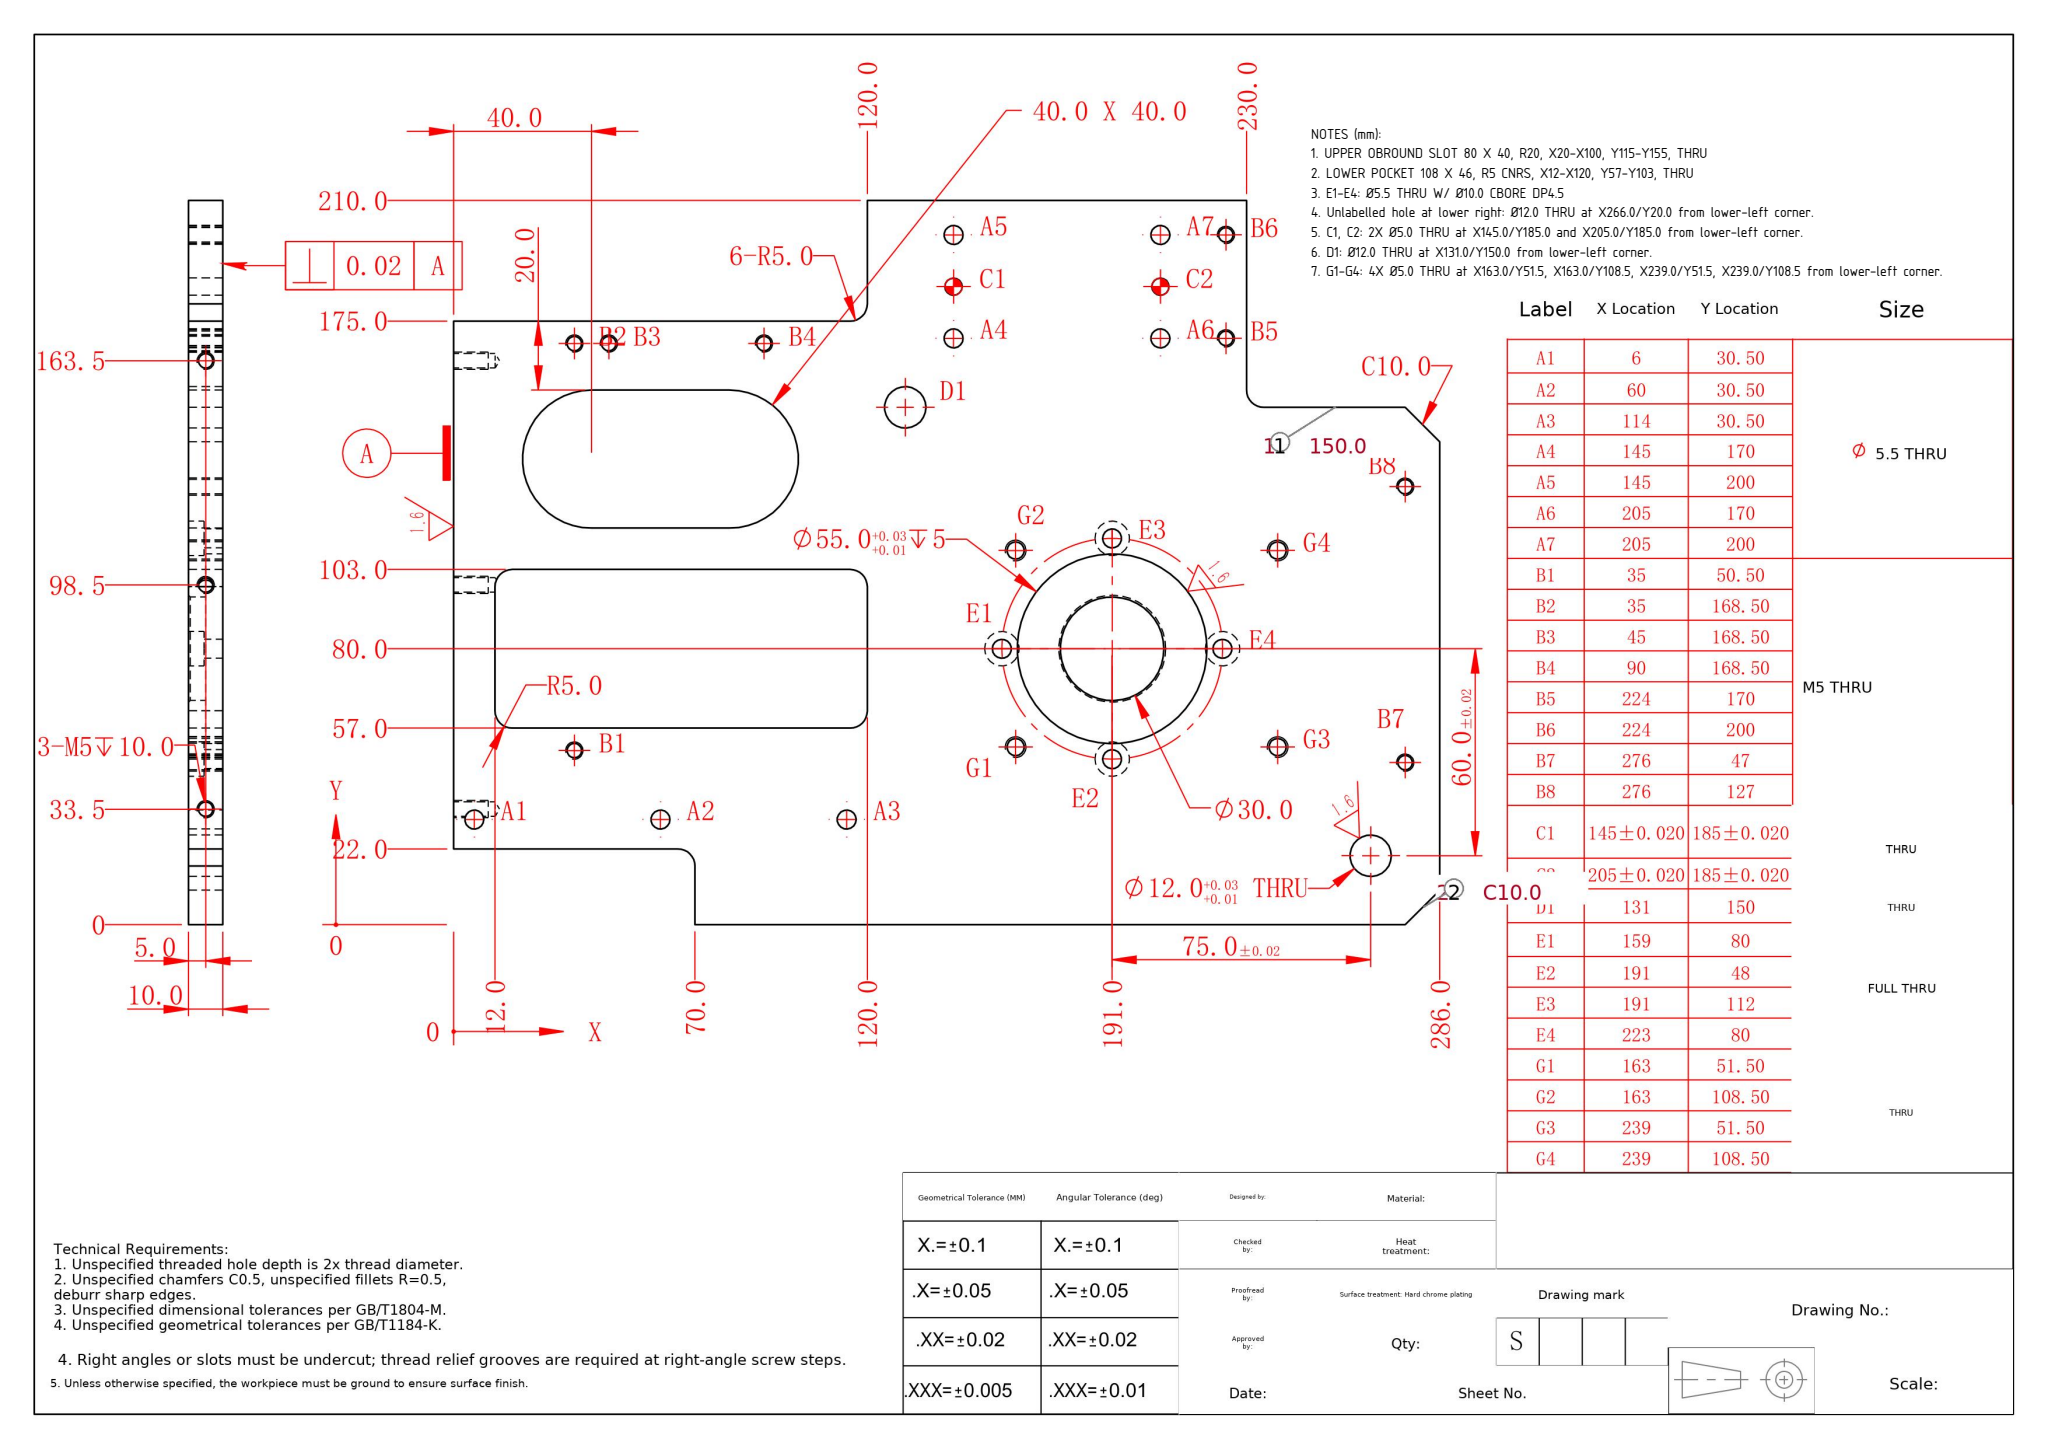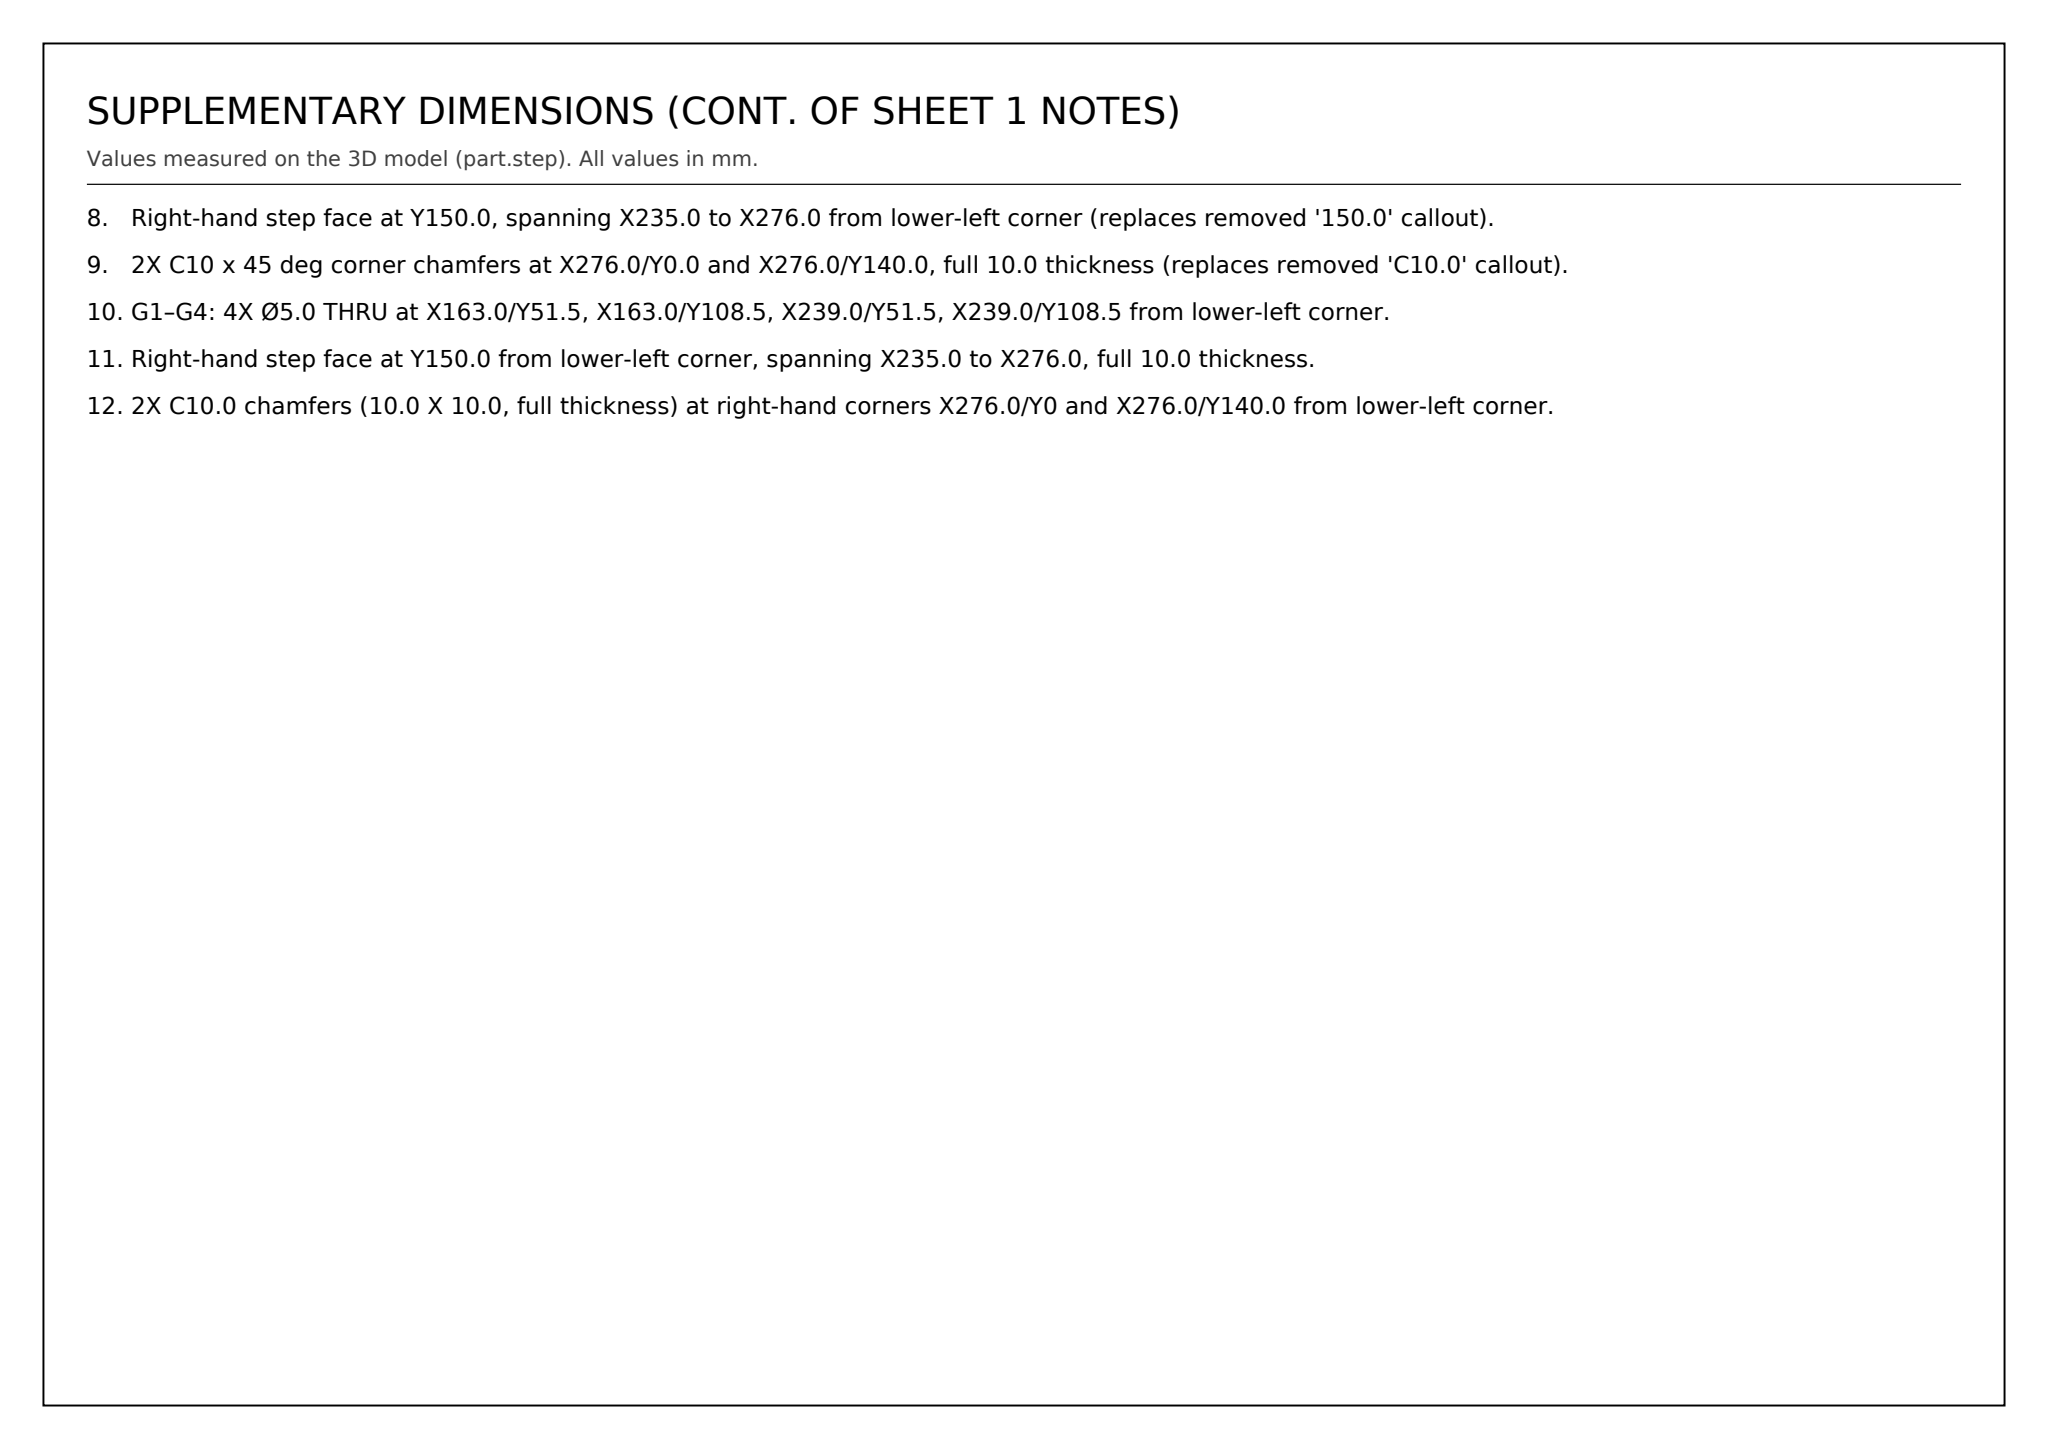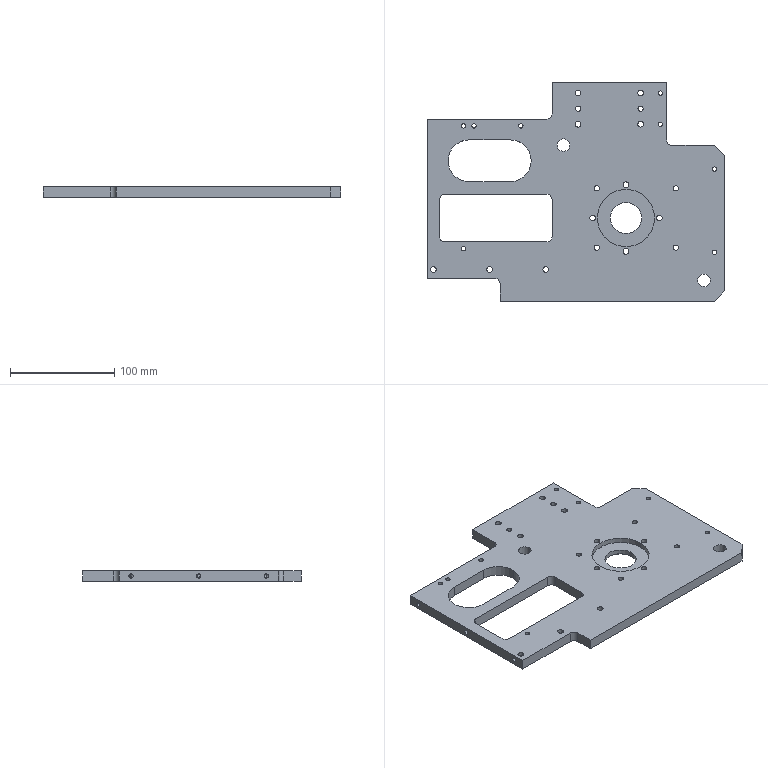Part | SolidWorks | mm | 1 solid | 116 faces | box 286 x 210 x 10 mm | volume 406665 mm3 | cylinder 82 | plane 25 | cone 9 | commonest cylinder face diameters 5.5 x22 4.2 x22 10 x15 5 x12 12 x4 40 x3 55 x2 30 x2
Drawing notes:
UPPER OBROUND SLOT 80 X 40, R20, X20-X100, Y115-Y155, THRU | from the solid: Ø40 cyls @ (40,135)&(80,135) len 10; planes y=115, y=155
LOWER POCKET 108 X 46, R5 CNRS, X12-X120, Y57-Y103, THRU | from the solid: R5 cnr cyls @ (17,62)(17,98)(115,62)(115,98) len 10; planes x=12/120, y=57/103
E1-E4: Ø5.5 THRU W/ Ø10.0 CBORE DP4.5 | from the solid: Ø5.5 len 5.5 and Ø10 len 4.5 coaxial @ (159,80)(191,48)(191,112)(223,80)
Unlabelled hole at lower right: Ø12.0 THRU at X266.0/Y20.0 from lower-left corner. | from the solid: cylinder dia 12.0, axis z, pos [266.0,20.0], length 10.0 = full 10.0 thk
C1, C2: 2X Ø5.0 THRU at X145.0/Y185.0 and X205.0/Y185.0 from lower-left corner. | from the solid: cylinders hole/bore dia 5.0, axis z at [145.0,185.0] and [205.0,185.0], from 0.0 to 10.0 (full 10 mm thickness)
D1: Ø12.0 THRU at X131.0/Y150.0 from lower-left corner. | from the solid: cylinders hole/bore dia 12.0, axis z at [131.0,150.0], from 0.0 to 10.0
G1-G4: 4X Ø5.0 THRU at X163.0/Y51.5, X163.0/Y108.5, X239.0/Y51.5, X239.0/Y108.5 from lower-left corner. | from the solid: cylinders hole/bore dia 5.0, axis z at [163.0,51.5], [163.0,108.5], [239.0,51.5], [239.0,108.5], from 0.0 to 10.0
Right-hand step face at Y150.0, spanning X235.0 to X276.0 from lower-left corner (replaces removed '150.0' callout). | from the solid: axis_planes normal y, offset 150.0, extent x [235.0,276.0], z [0.0,10.0]
2X C10 x 45 deg corner chamfers at X276.0/Y0.0 and X276.0/Y140.0, full 10.0 thickness (replaces removed 'C10.0' callout). | from the solid: inclined_planes 45/45/90 deg, bbox_from [276.0,0.0,0.0] and [276.0,140.0,0.0], size 10x10x10
G1–G4: 4X Ø5.0 THRU at X163.0/Y51.5, X163.0/Y108.5, X239.0/Y51.5, X239.0/Y108.5 from lower-left corner. | from the solid: cylinders hole/bore dia 5.0 axis z at [163.0,51.5], [163.0,108.5], [239.0,51.5], [239.0,108.5], from 0.0 to 10.0
Right-hand step face at Y150.0 from lower-left corner, spanning X235.0 to X276.0, full 10.0 thickness. | from the solid: axis_planes normal y, offset 150.0, extent x [235.0,276.0], z [0.0,10.0]
2X C10.0 chamfers (10.0 X 10.0, full thickness) at right-hand corners X276.0/Y0 and X276.0/Y140.0 from lower-left corner. | from the solid: inclined_planes 45°/45°/90° bbox_from [276.0,0.0,0.0] and [276.0,140.0,0.0], size [10.0,10.0,10.0]
build123d program:
from build123d import *

# Parameters (mm, degrees)
SKETCH1_W                                            = 286
SKETCH1_H                                            = 210
BOSS_EXTRUDE1_DEPTH                                  = 5
CUT_EXTRUDE1_REACH                                   = 179.691
SKETCH2_W                                            = 120
SKETCH2_H                                            = 35
SKETCH2_W_2                                          = 56
SKETCH2_H_2                                          = 60
SKETCH2_W_3                                          = 70
SKETCH2_H_3                                          = 22
CUT_EXTRUDE2_REACH                                   = 179.691
SKETCH3_W                                            = 108
SKETCH3_H                                            = 46
FILLET1_R                                            = 5
CUT_EXTRUDE3_REACH                                   = 179.691
SKETCH4_R                                            = 15
SKETCH4_R_2                                          = 6
M5_TAPPED_HOLE1_D                                    = 4.2
F_5_5_5_5_DIAMETER_HOLE1_D                           = 5.5
F_5_0_5_DIAMETER_HOLE1_D                             = 5
M6_TAPPED_HOLE2_D                                    = 5
M5_TAPPED_HOLE2_D                                    = 4.2
M5_TAPPED_HOLE2_DEPTH                                = 12
M5_TAPPED_HOLE2_TIP                                  = 1.262
CHAMFER1_SIZE                                        = 0.5
CHAMFER2_SIZE                                        = 10
SKETCH15_R                                           = 27.5
CUT_EXTRUDE4_DEPTH                                   = 5
HOLE_SIZE_ACCORDING_TO_THE_TYPE_OF_HEXAG_D           = 5.5
HOLE_SIZE_ACCORDING_TO_THE_TYPE_OF_HEXAG_CBORE_D     = 10
HOLE_SIZE_ACCORDING_TO_THE_TYPE_OF_HEXAG_CBORE_DEPTH = 4.5
CIRPATTERN1_COUNT                                    = 4
CUT_EXTRUDE5_DEPTH                                   = 178.691


with BuildPart() as part:
    # Sketch1 → Boss-Extrude1 (new, symmetric)
    with BuildSketch(Plane.XY):
        Rectangle(SKETCH1_W, SKETCH1_H)
    extrude(amount=BOSS_EXTRUDE1_DEPTH, both=True)

    # Sketch2 → Cut-Extrude1 (cut, up to next)
    with BuildSketch(Plane.XY.offset(5), mode=Mode.PRIVATE) as cut_extrude1_sk1:
        with Locations((-83, 87.5)):
            Rectangle(SKETCH2_W, SKETCH2_H)
    cut_extrude1_tool1 = extrude(cut_extrude1_sk1.sketch, amount=-CUT_EXTRUDE1_REACH, mode=Mode.PRIVATE) & part.part
    # Sketch2 → Cut-Extrude1 (cut, up to next)
    with BuildSketch(Plane.XY.offset(5), mode=Mode.PRIVATE) as cut_extrude1_sk2:
        with Locations((115, 75)):
            Rectangle(SKETCH2_W_2, SKETCH2_H_2)
    cut_extrude1_tool2 = extrude(cut_extrude1_sk2.sketch, amount=-CUT_EXTRUDE1_REACH, mode=Mode.PRIVATE) & part.part
    # Sketch2 → Cut-Extrude1 (cut, up to next)
    with BuildSketch(Plane.XY.offset(5), mode=Mode.PRIVATE) as cut_extrude1_sk3:
        with Locations((-108, -94)):
            Rectangle(SKETCH2_W_3, SKETCH2_H_3)
    cut_extrude1_tool3 = extrude(cut_extrude1_sk3.sketch, amount=-CUT_EXTRUDE1_REACH, mode=Mode.PRIVATE) & part.part
    add(cut_extrude1_tool1.solids().sort_by_distance((-83, 87.5, 5))[0], mode=Mode.SUBTRACT)
    add(cut_extrude1_tool2.solids().sort_by_distance((115, 75, 5))[0], mode=Mode.SUBTRACT)
    add(cut_extrude1_tool3.solids().sort_by_distance((-108, -94, 5))[0], mode=Mode.SUBTRACT)

    # Sketch3 → Cut-Extrude2 (cut, up to next)
    with BuildSketch(Plane.XY.offset(5), mode=Mode.PRIVATE) as cut_extrude2_sk1:
        with Locations((-77, -25)):
            Rectangle(SKETCH3_W, SKETCH3_H)
    cut_extrude2_tool1 = extrude(cut_extrude2_sk1.sketch, amount=-CUT_EXTRUDE2_REACH, mode=Mode.PRIVATE) & part.part
    add(cut_extrude2_tool1.solids().sort_by_distance((-77, -25, 5))[0], mode=Mode.SUBTRACT)

    # Fillet1
    fillet1_edges = [part.edges().sort_by_distance(p)[0] for p in [
        (-23, 70, 0),
        (87, 45, 0),
        (-73, -83, 0),
        (-131, -48, 0),
        (-131, -2, 0),
        (-23, -2, 0),
        (-23, -48, 0),
    ]]
    fillet(fillet1_edges, radius=FILLET1_R)

    # Sketch4 → Cut-Extrude3 (cut, up to next)
    with BuildSketch(Plane.XY.offset(5), mode=Mode.PRIVATE) as cut_extrude3_sk1:
        with Locations((48, -25)):
            Circle(SKETCH4_R)
    cut_extrude3_tool1 = extrude(cut_extrude3_sk1.sketch, amount=-CUT_EXTRUDE3_REACH, mode=Mode.PRIVATE) & part.part
    # Sketch4 → Cut-Extrude3 (cut, up to next)
    with BuildSketch(Plane.XY.offset(5), mode=Mode.PRIVATE) as cut_extrude3_sk2:
        with Locations((-12, 45)):
            Circle(SKETCH4_R_2)
    cut_extrude3_tool2 = extrude(cut_extrude3_sk2.sketch, amount=-CUT_EXTRUDE3_REACH, mode=Mode.PRIVATE) & part.part
    # Sketch4 → Cut-Extrude3 (cut, up to next)
    with BuildSketch(Plane.XY.offset(5), mode=Mode.PRIVATE) as cut_extrude3_sk3:
        with Locations((123, -85)):
            Circle(SKETCH4_R_2)
    cut_extrude3_tool3 = extrude(cut_extrude3_sk3.sketch, amount=-CUT_EXTRUDE3_REACH, mode=Mode.PRIVATE) & part.part
    add(cut_extrude3_tool1.solids().sort_by_distance((48, -25, 5))[0], mode=Mode.SUBTRACT)
    add(cut_extrude3_tool2.solids().sort_by_distance((-12, 45, 5))[0], mode=Mode.SUBTRACT)
    add(cut_extrude3_tool3.solids().sort_by_distance((123, -85, 5))[0], mode=Mode.SUBTRACT)

    # M5 Tapped Hole1 (through all)
    with Locations(Plane.XY.offset(5)):
        with Locations((81, 95), (81, 65), (133, 22), (133, -58), (-108, 63.5), (-98, 63.5), (-53, 63.5), (-108, -54.5)):
            Hole(M5_TAPPED_HOLE1_D / 2)

    # 5.5 _5.5_ Diameter Hole1 (through all)
    with Locations(Plane.XY.offset(5)):
        with Locations((-29, -74.5), (-137, -74.5), (2, 95), (2, 65), (62, 95), (62, 65), (-83, -74.5)):
            Hole(F_5_5_5_5_DIAMETER_HOLE1_D / 2)

    # 5.0 _5_ Diameter Hole1 (through all)
    with Locations(Plane.XY.offset(5)):
        with Locations((2, 80), (62, 80)):
            Hole(F_5_0_5_DIAMETER_HOLE1_D / 2)

    # M6 Tapped Hole2 (through all)
    with Locations(Plane.XY.offset(5)):
        with Locations((20, 3.5), (96, -53.5), (20, -53.5), (96, 3.5)):
            Hole(M6_TAPPED_HOLE2_D / 2)

    # M5 Tapped Hole2
    with Locations(Plane.ZY.offset(143)):
        with Locations((0, 58.5), (0, -6.5), (0, -71.5)):
            Hole(M5_TAPPED_HOLE2_D / 2, depth=M5_TAPPED_HOLE2_DEPTH)
            with Locations((0, 0, -(M5_TAPPED_HOLE2_DEPTH + M5_TAPPED_HOLE2_TIP / 2))):  # 118° drill point
                Cone(0, M5_TAPPED_HOLE2_D / 2, M5_TAPPED_HOLE2_TIP, mode=Mode.SUBTRACT)

    # Chamfer1
    chamfer1_edges = [part.edges().sort_by_distance(p)[0] for p in [
        (33, -25, 5),
        (33, -25, -5),
    ]]
    chamfer(chamfer1_edges, length=CHAMFER1_SIZE)

    # Chamfer2
    chamfer2_edges = [part.edges().sort_by_distance(p)[0] for p in [
        (143, 45, 0),
        (143, -105, 0),
    ]]
    chamfer(chamfer2_edges, length=CHAMFER2_SIZE)

    # Sketch15 → Cut-Extrude4 (cut)
    with BuildSketch(Plane.XY.offset(5)):
        with Locations((48, -25)):
            Circle(SKETCH15_R)
    extrude(amount=-CUT_EXTRUDE4_DEPTH, mode=Mode.SUBTRACT)

    # Hole Size according to the type of Hexag (through all)
    with Locations(Plane(origin=(0, 0, -5), x_dir=(-1, 0, 0), z_dir=(0, 0, -1))):
        with Locations((-80, -25)):
            hole_size_according_to_the_type_of_hexag = CounterBoreHole(HOLE_SIZE_ACCORDING_TO_THE_TYPE_OF_HEXAG_D / 2, HOLE_SIZE_ACCORDING_TO_THE_TYPE_OF_HEXAG_CBORE_D / 2, HOLE_SIZE_ACCORDING_TO_THE_TYPE_OF_HEXAG_CBORE_DEPTH)

    # CirPattern1: Hole Size according to the type of Hexag ×4 about axis
    cirpattern1_axis = Axis((48, -25, 0), (0, 0, 1))
    for i in range(1, CIRPATTERN1_COUNT):
        add(hole_size_according_to_the_type_of_hexag.rotate(cirpattern1_axis, i * 360 / CIRPATTERN1_COUNT), mode=Mode.SUBTRACT)

    # Sketch18 → Cut-Extrude5 (cut, through all)
    with BuildSketch(Plane.XY.offset(5)):
        with BuildLine():
            Line((-103, 50), (-63, 50))
            ThreePointArc((-63, 50), (-43, 30), (-63, 10))
            Line((-63, 10), (-103, 10))
            ThreePointArc((-103, 10), (-123, 30), (-103, 50))
        make_face()
    extrude(amount=-CUT_EXTRUDE5_DEPTH, mode=Mode.SUBTRACT)


solid = part.part